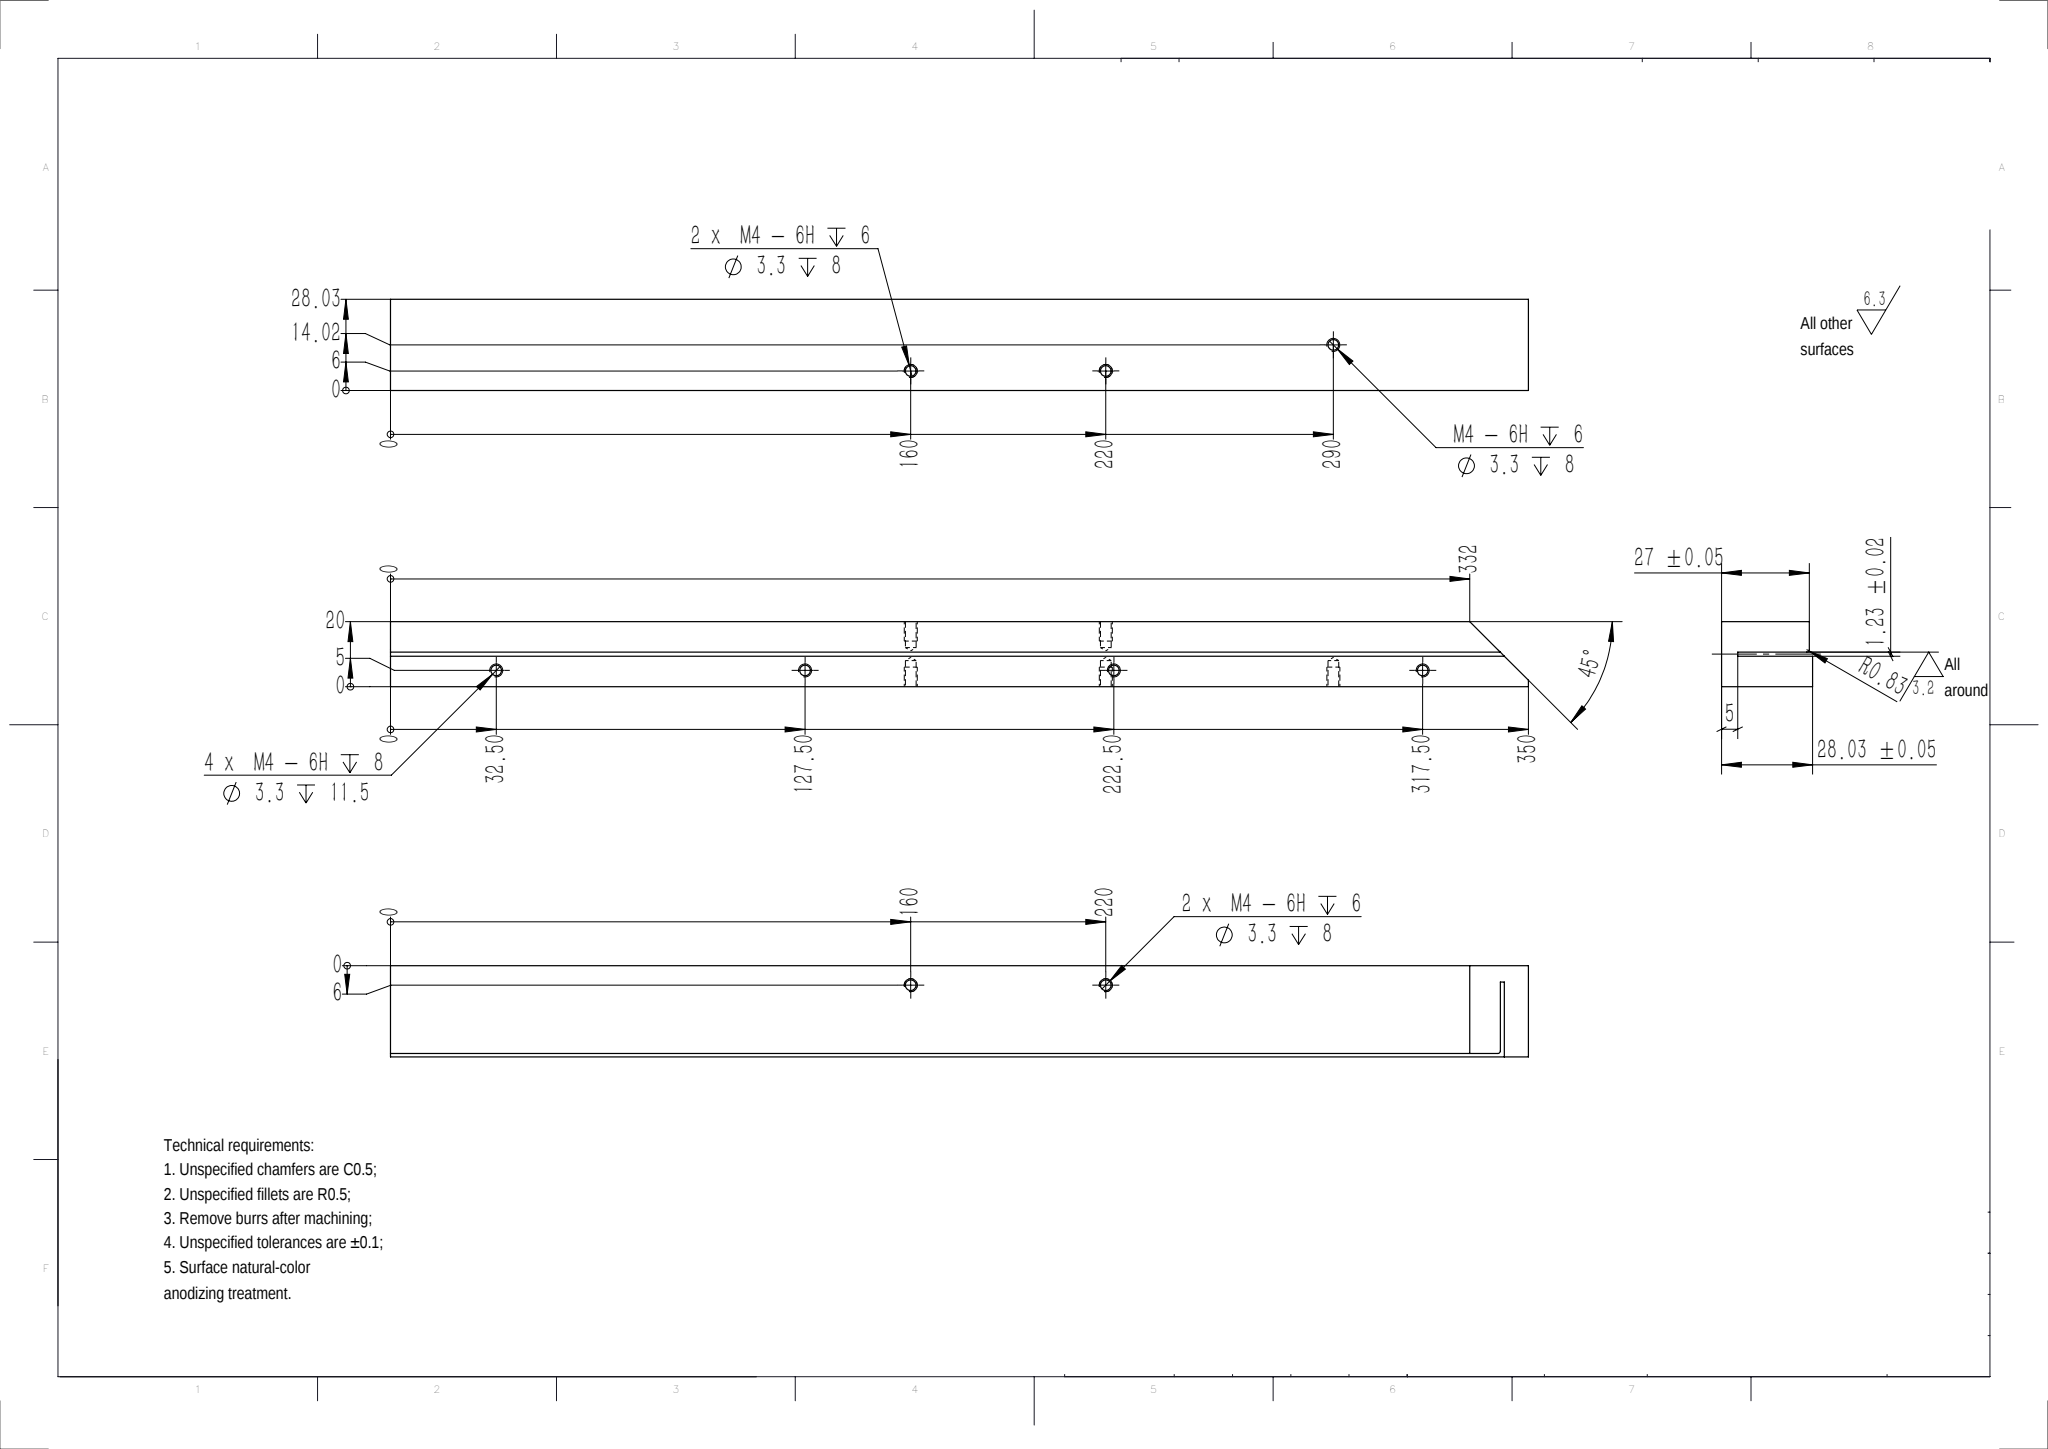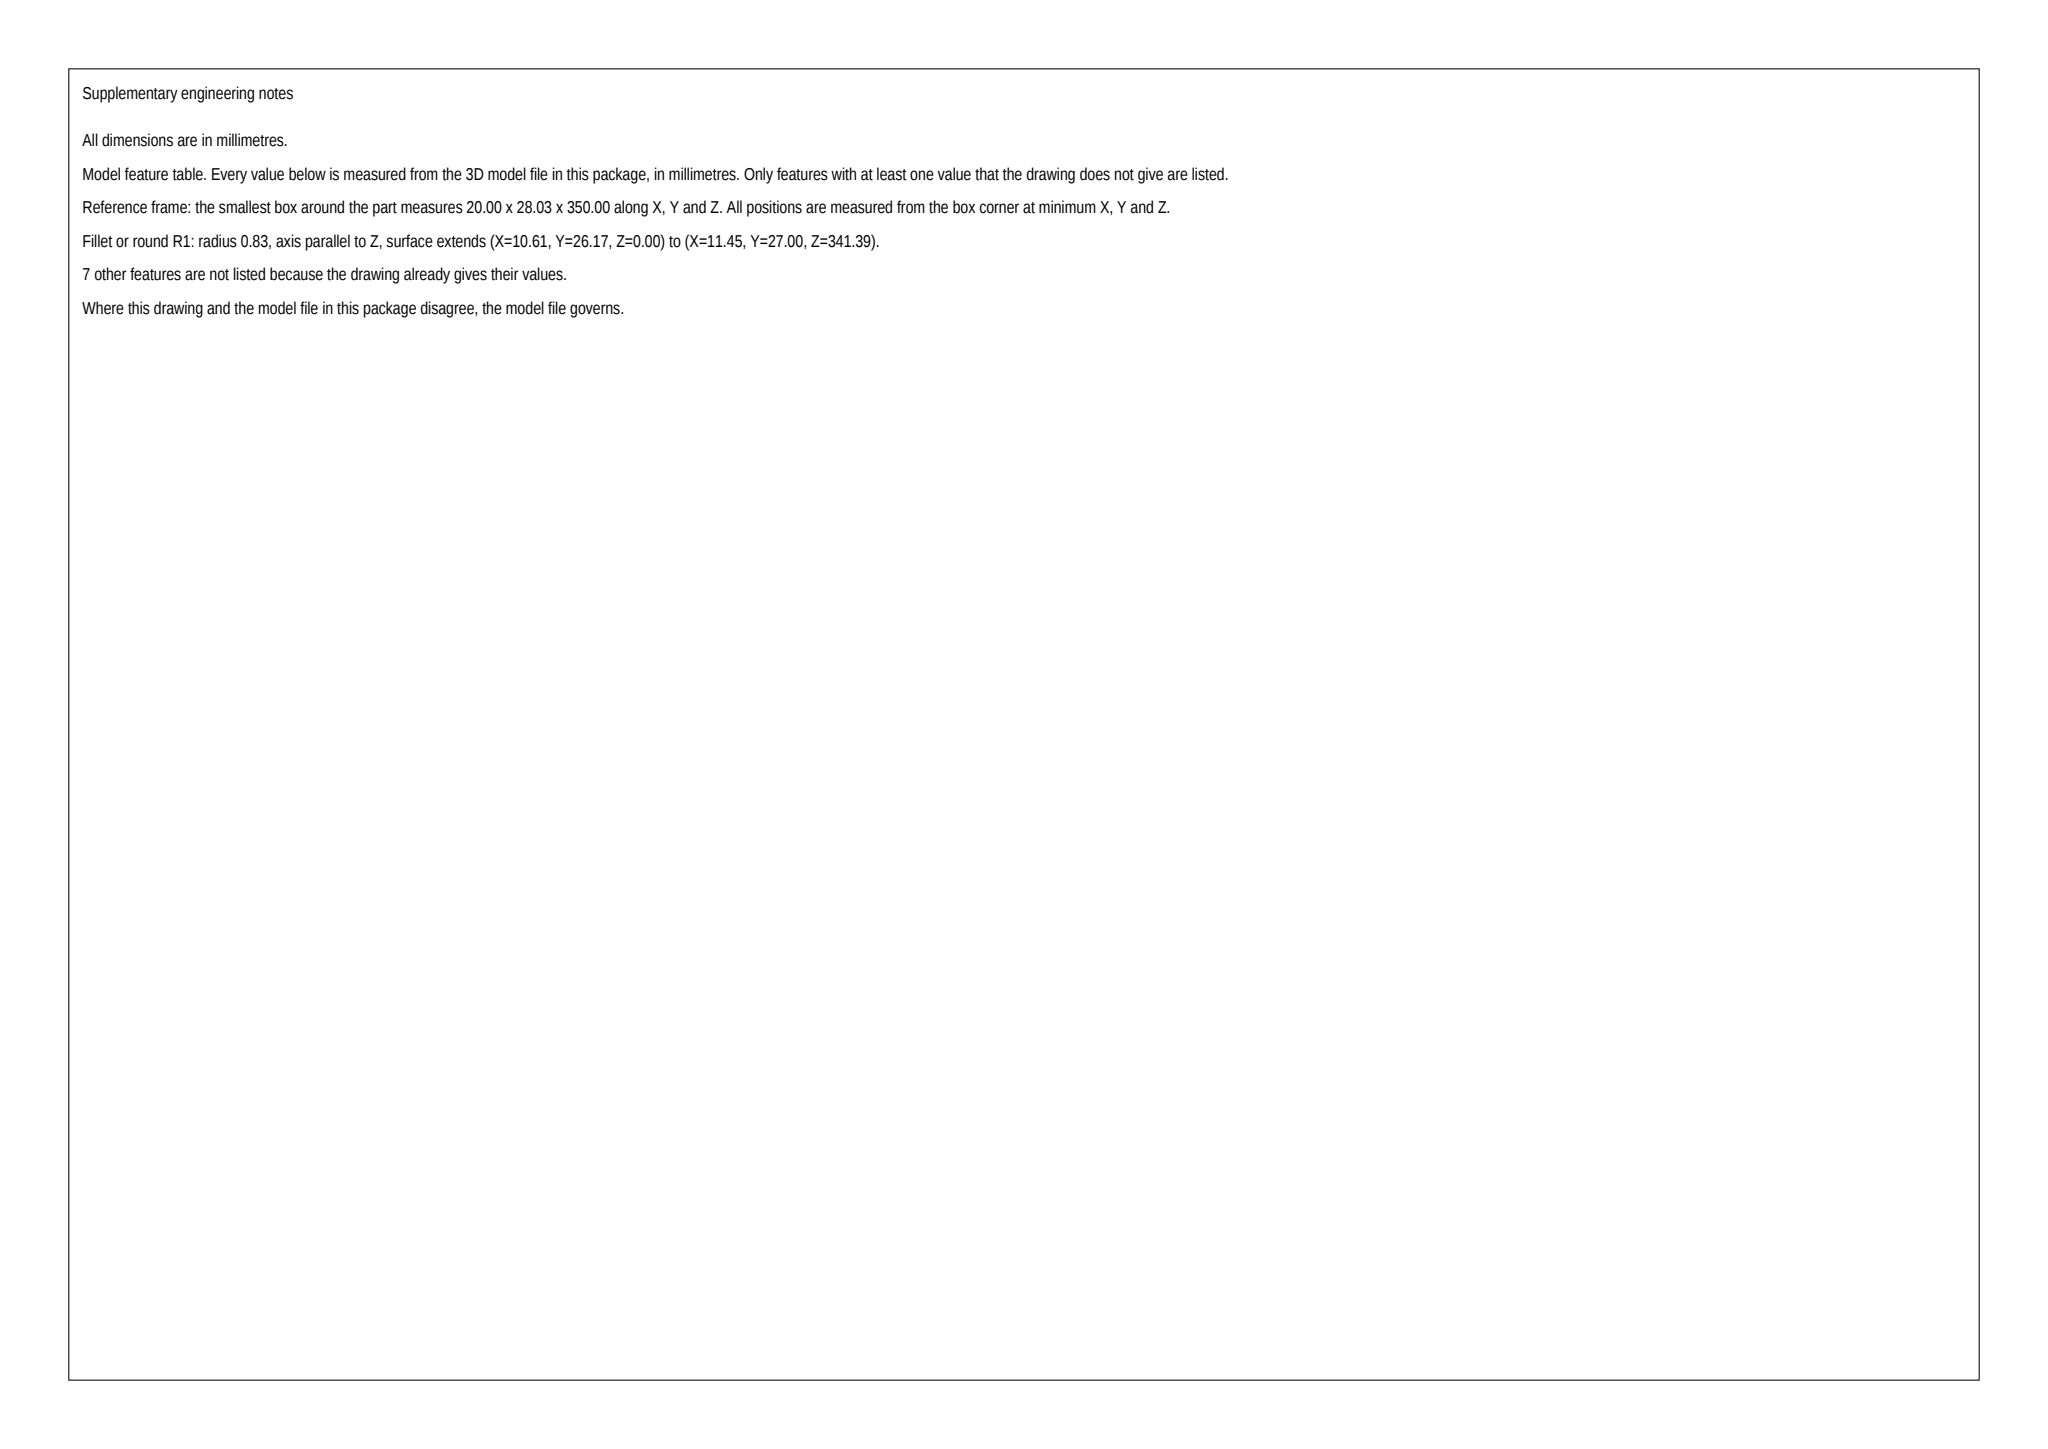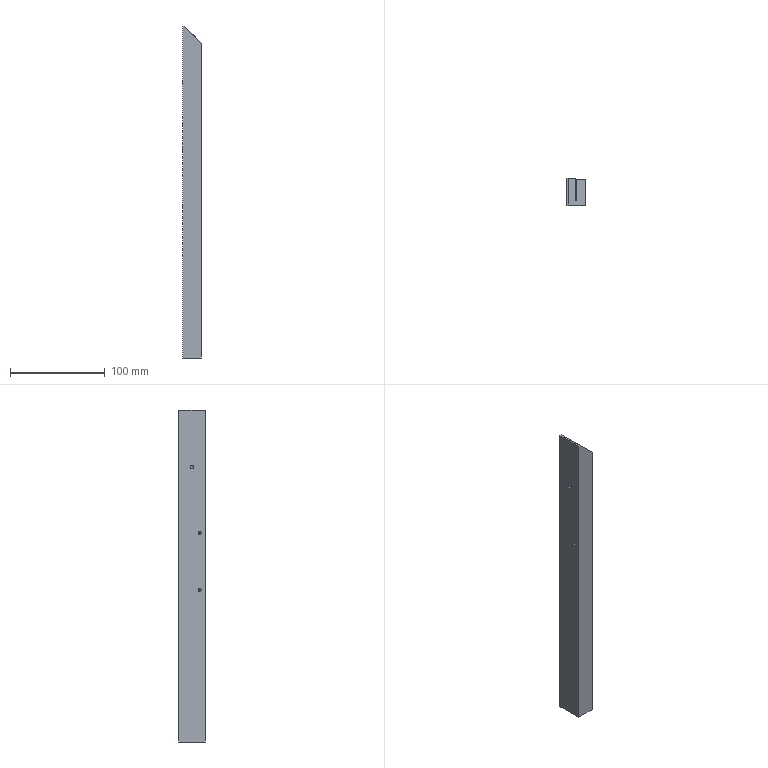Part | SolidWorks | mm | 1 solid | 48 faces | box 20 x 28.03 x 350 mm | volume 177915 mm3 | cylinder 19 | cone 18 | plane 11 | commonest cylinder face diameters 3.3 x18 1.66 x1
build123d program:
from build123d import *

# Parameters (mm, degrees)
BOSS_EXTRUDE1_DEPTH        = 350
FILLET1_R                  = 0.83
M4_TAPPED_HOLE1_D          = 3.3
M4_TAPPED_HOLE1_DEPTH      = 11.5
M4_TAPPED_HOLE1_TIP        = 0.9914
M4_TAPPED_HOLE2_AT_2_COUNT = 2
M4_TAPPED_HOLE2_AT_2_PITCH = 60
M4_TAPPED_HOLE3_D          = 3.3
M4_TAPPED_HOLE3_DEPTH      = 8
M4_TAPPED_HOLE3_TIP        = 0.9914
CUT_EXTRUDE1_DEPTH         = 352.263


with BuildPart() as part:
    # Sketch1 → Boss-Extrude1 (new body)
    with BuildSketch(Plane.XY):
        Polygon((-10, 0), (10, 0), (10, 27), (0.615, 27), (0.615, 5), (-0.615, 5), (-0.615, 28.03), (-10, 28.03), align=None)
    extrude(amount=BOSS_EXTRUDE1_DEPTH)

    # Fillet1
    fillet1_edges = [part.edges().sort_by_distance(p)[0] for p in [
        (0.615, 27, 175),
    ]]
    fillet(fillet1_edges, radius=FILLET1_R)

    # M4 Tapped Hole1
    with Locations(Plane(origin=(0, 28.03, 0), x_dir=(1, 0, 0), z_dir=(0, 1, 0))):
        with Locations((-5, -317.5), (-5, -222.5), (-5, -127.5), (-5, -32.5)):
            Hole(M4_TAPPED_HOLE1_D / 2, depth=M4_TAPPED_HOLE1_DEPTH)
            with Locations((0, 0, -(M4_TAPPED_HOLE1_DEPTH + M4_TAPPED_HOLE1_TIP / 2))):  # 118° drill point
                Cone(0, M4_TAPPED_HOLE1_D / 2, M4_TAPPED_HOLE1_TIP, mode=Mode.SUBTRACT)

    # Sketch6 → M4 Tapped Hole2 (revolve, cut)
    with BuildSketch(Plane(origin=(10, 6, 220), x_dir=(0, 0, -1), z_dir=(0, 1, 0))):
        Polygon((0, 0), (0, 8.991), (1.65, 8), (1.65, 0), align=None)
    m4_tapped_hole2 = revolve(axis=Axis((16.35, 6, 220), (-1, 0, 0)), mode=Mode.SUBTRACT)

    # M4 Tapped Hole2 at 2: M4 Tapped Hole2 ×2
    with Locations(*[(0, 0, -i * M4_TAPPED_HOLE2_AT_2_PITCH) for i in range(1, M4_TAPPED_HOLE2_AT_2_COUNT)]):
        add(m4_tapped_hole2, mode=Mode.SUBTRACT)

    # Mirror1: M4 Tapped Hole2 across plane
    add(m4_tapped_hole2.mirror(Plane(origin=(0, 0, 0), x_dir=(0, 0, 1), z_dir=(1, 0, 0))), mode=Mode.SUBTRACT)

    # Mirror1 copy 1 sketch → Mirror1 copy 1 (revolve, cut)
    with BuildSketch(Plane(origin=(-10, 6, 160), x_dir=(0, 0, -1), z_dir=(0, 1, 0))):
        Polygon((0, 0), (0, -8.991), (1.65, -8), (1.65, 0), align=None)
    revolve(axis=Axis((-16.35, 6, 160), (-1, 0, 0)), mode=Mode.SUBTRACT)

    # M4 Tapped Hole3
    with Locations(Plane.ZY.offset(10)):
        with Locations((290, 14.015)):
            Hole(M4_TAPPED_HOLE3_D / 2, depth=M4_TAPPED_HOLE3_DEPTH)
            with Locations((0, 0, -(M4_TAPPED_HOLE3_DEPTH + M4_TAPPED_HOLE3_TIP / 2))):  # 118° drill point
                Cone(0, M4_TAPPED_HOLE3_D / 2, M4_TAPPED_HOLE3_TIP, mode=Mode.SUBTRACT)

    # Sketch10 → Cut-Extrude1 (cut, through all)
    with BuildSketch(Plane(origin=(0, 28.03, 0), x_dir=(1, 0, 0), z_dir=(0, 1, 0))):
        Polygon((-8, -350), (10, -332), (10, -350), align=None)
    extrude(amount=-CUT_EXTRUDE1_DEPTH, mode=Mode.SUBTRACT)


solid = part.part